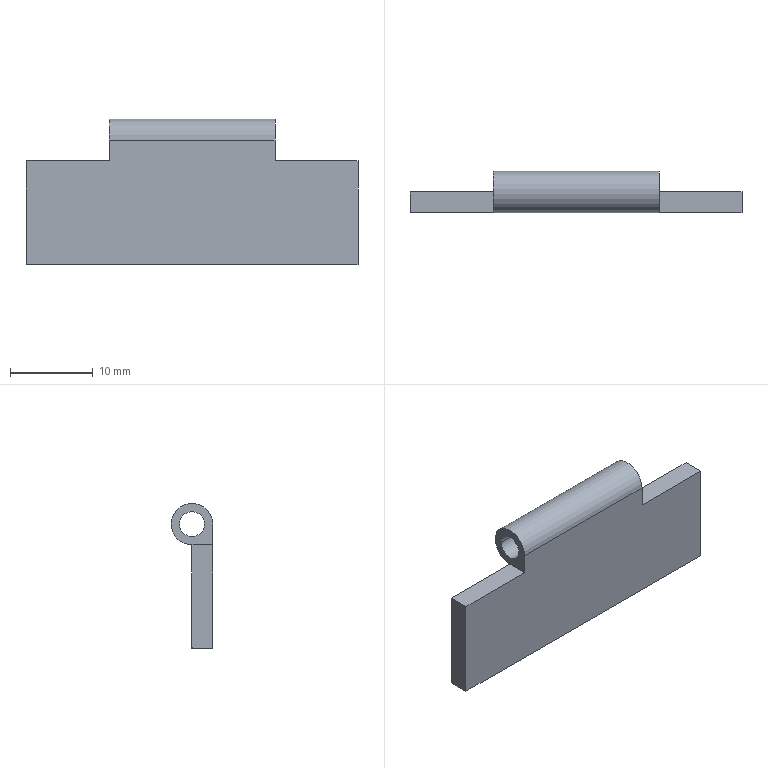Component | SolidWorks | ButtonStation-1_Hinge2-1 | 1 solid | 13 faces | box 40 x 5 x 17.5 mm | volume 1528 mm3 | plane 9 | cylinder 4 | commonest cylinder face diameters 5 x2 3 x2 | material Plain Carbon Steel
STEP:
#1=COLOUR_RGB('',0.7922,0.8196,0.9333);
#2=FILL_AREA_STYLE_COLOUR('',#1);
#3=FILL_AREA_STYLE('',(#2));
#4=SURFACE_STYLE_FILL_AREA(#3);
#5=SURFACE_SIDE_STYLE('',(#4));
#6=SURFACE_STYLE_USAGE(.BOTH.,#5);
#7=PRESENTATION_STYLE_ASSIGNMENT((#6));
#8=CARTESIAN_POINT('',(6.339,24.705,26.713));
#9=VERTEX_POINT('',#8);
#10=CARTESIAN_POINT('',(6.339,24.902,26.713));
#11=VERTEX_POINT('',#10);
#12=CARTESIAN_POINT('',(6.339,24.803,26.713));
#13=DIRECTION('',(-1.,-0.,-0.));
#14=DIRECTION('',(0.,1.,0.));
#15=AXIS2_PLACEMENT_3D('',#12,#13,#14);
#16=CIRCLE('',#15,0.09843);
#17=EDGE_CURVE('',#9,#11,#16,.T.);
#18=ORIENTED_EDGE('',*,*,#17,.T.);
#19=CARTESIAN_POINT('',(5.551,24.902,26.713));
#20=VERTEX_POINT('',#19);
#21=CARTESIAN_POINT('',(6.732,24.902,26.713));
#22=DIRECTION('',(-1.,-0.,-0.));
#23=VECTOR('',#22,39.37);
#24=LINE('',#21,#23);
#25=EDGE_CURVE('',#11,#20,#24,.T.);
#26=ORIENTED_EDGE('',*,*,#25,.T.);
#27=CARTESIAN_POINT('',(5.551,24.705,26.713));
#28=VERTEX_POINT('',#27);
#29=CARTESIAN_POINT('',(5.551,24.803,26.713));
#30=DIRECTION('',(1.,0.,0.));
#31=DIRECTION('',(0.,1.,0.));
#32=AXIS2_PLACEMENT_3D('',#29,#30,#31);
#33=CIRCLE('',#32,0.09843);
#34=EDGE_CURVE('',#20,#28,#33,.T.);
#35=ORIENTED_EDGE('',*,*,#34,.T.);
#36=CARTESIAN_POINT('',(6.732,24.705,26.713));
#37=DIRECTION('',(-1.,-0.,-0.));
#38=VECTOR('',#37,39.37);
#39=LINE('',#36,#38);
#40=EDGE_CURVE('',#9,#28,#39,.T.);
#41=ORIENTED_EDGE('',*,*,#40,.F.);
#42=EDGE_LOOP('',(#18,#26,#35,#41));
#43=FACE_OUTER_BOUND('',#42,.T.);
#44=CARTESIAN_POINT('',(6.732,24.803,26.713));
#45=DIRECTION('',(-1.,-0.,-0.));
#46=DIRECTION('',(0.,1.,0.));
#47=AXIS2_PLACEMENT_3D('',#44,#45,#46);
#48=CYLINDRICAL_SURFACE('',#47,0.09843);
#49=ADVANCED_FACE('',(#43),#48,.T.);
#50=CARTESIAN_POINT('',(6.339,24.862,26.713));
#51=VERTEX_POINT('',#50);
#52=CARTESIAN_POINT('',(6.339,24.744,26.713));
#53=VERTEX_POINT('',#52);
#54=CARTESIAN_POINT('',(6.339,24.803,26.713));
#55=DIRECTION('',(1.,0.,0.));
#56=DIRECTION('',(0.,1.,0.));
#57=AXIS2_PLACEMENT_3D('',#54,#55,#56);
#58=CIRCLE('',#57,0.05906);
#59=EDGE_CURVE('',#51,#53,#58,.T.);
#60=ORIENTED_EDGE('',*,*,#59,.T.);
#61=CARTESIAN_POINT('',(5.551,24.744,26.713));
#62=VERTEX_POINT('',#61);
#63=CARTESIAN_POINT('',(6.732,24.744,26.713));
#64=DIRECTION('',(-1.,-0.,-0.));
#65=VECTOR('',#64,39.37);
#66=LINE('',#63,#65);
#67=EDGE_CURVE('',#53,#62,#66,.T.);
#68=ORIENTED_EDGE('',*,*,#67,.T.);
#69=CARTESIAN_POINT('',(5.551,24.862,26.713));
#70=VERTEX_POINT('',#69);
#71=CARTESIAN_POINT('',(5.551,24.803,26.713));
#72=DIRECTION('',(-1.,-0.,-0.));
#73=DIRECTION('',(0.,1.,0.));
#74=AXIS2_PLACEMENT_3D('',#71,#72,#73);
#75=CIRCLE('',#74,0.05906);
#76=EDGE_CURVE('',#62,#70,#75,.T.);
#77=ORIENTED_EDGE('',*,*,#76,.T.);
#78=CARTESIAN_POINT('',(6.732,24.862,26.713));
#79=DIRECTION('',(-1.,-0.,-0.));
#80=VECTOR('',#79,39.37);
#81=LINE('',#78,#80);
#82=EDGE_CURVE('',#51,#70,#81,.T.);
#83=ORIENTED_EDGE('',*,*,#82,.F.);
#84=EDGE_LOOP('',(#60,#68,#77,#83));
#85=FACE_OUTER_BOUND('',#84,.T.);
#86=CARTESIAN_POINT('',(6.732,24.803,26.713));
#87=DIRECTION('',(-1.,-0.,-0.));
#88=DIRECTION('',(0.,1.,0.));
#89=AXIS2_PLACEMENT_3D('',#86,#87,#88);
#90=CYLINDRICAL_SURFACE('',#89,0.05906);
#91=ADVANCED_FACE('',(#85),#90,.F.);
#92=CARTESIAN_POINT('',(6.339,24.705,26.614));
#93=VERTEX_POINT('',#92);
#94=CARTESIAN_POINT('',(6.339,24.705,27.065));
#95=DIRECTION('',(-0.,0.,1.));
#96=VECTOR('',#95,39.37);
#97=LINE('',#94,#96);
#98=EDGE_CURVE('',#93,#9,#97,.T.);
#99=ORIENTED_EDGE('',*,*,#98,.T.);
#100=ORIENTED_EDGE('',*,*,#40,.T.);
#101=CARTESIAN_POINT('',(5.551,24.705,26.614));
#102=VERTEX_POINT('',#101);
#103=CARTESIAN_POINT('',(5.551,24.705,27.065));
#104=DIRECTION('',(0.,-0.,-1.));
#105=VECTOR('',#104,39.37);
#106=LINE('',#103,#105);
#107=EDGE_CURVE('',#28,#102,#106,.T.);
#108=ORIENTED_EDGE('',*,*,#107,.T.);
#109=CARTESIAN_POINT('',(5.157,24.705,26.614));
#110=VERTEX_POINT('',#109);
#111=CARTESIAN_POINT('',(6.732,24.705,26.614));
#112=DIRECTION('',(-1.,-0.,-0.));
#113=VECTOR('',#112,39.37);
#114=LINE('',#111,#113);
#115=EDGE_CURVE('',#102,#110,#114,.T.);
#116=ORIENTED_EDGE('',*,*,#115,.T.);
#117=CARTESIAN_POINT('',(5.157,24.705,26.122));
#118=VERTEX_POINT('',#117);
#119=CARTESIAN_POINT('',(5.157,24.705,27.065));
#120=DIRECTION('',(0.,-0.,-1.));
#121=VECTOR('',#120,39.37);
#122=LINE('',#119,#121);
#123=EDGE_CURVE('',#110,#118,#122,.T.);
#124=ORIENTED_EDGE('',*,*,#123,.T.);
#125=CARTESIAN_POINT('',(6.732,24.705,26.122));
#126=VERTEX_POINT('',#125);
#127=CARTESIAN_POINT('',(6.732,24.705,26.122));
#128=DIRECTION('',(1.,0.,0.));
#129=VECTOR('',#128,39.37);
#130=LINE('',#127,#129);
#131=EDGE_CURVE('',#118,#126,#130,.T.);
#132=ORIENTED_EDGE('',*,*,#131,.T.);
#133=CARTESIAN_POINT('',(6.732,24.705,26.614));
#134=VERTEX_POINT('',#133);
#135=CARTESIAN_POINT('',(6.732,24.705,27.065));
#136=DIRECTION('',(-0.,0.,1.));
#137=VECTOR('',#136,39.37);
#138=LINE('',#135,#137);
#139=EDGE_CURVE('',#126,#134,#138,.T.);
#140=ORIENTED_EDGE('',*,*,#139,.T.);
#141=CARTESIAN_POINT('',(6.732,24.705,26.614));
#142=DIRECTION('',(-1.,-0.,-0.));
#143=VECTOR('',#142,39.37);
#144=LINE('',#141,#143);
#145=EDGE_CURVE('',#134,#93,#144,.T.);
#146=ORIENTED_EDGE('',*,*,#145,.T.);
#147=EDGE_LOOP('',(#99,#100,#108,#116,#124,#132,#140,#146));
#148=FACE_OUTER_BOUND('',#147,.T.);
#149=CARTESIAN_POINT('',(6.732,24.705,27.065));
#150=DIRECTION('',(0.,-1.,0.));
#151=DIRECTION('',(-0.,0.,1.));
#152=AXIS2_PLACEMENT_3D('',#149,#150,#151);
#153=PLANE('',#152);
#154=ADVANCED_FACE('',(#148),#153,.T.);
#155=ORIENTED_EDGE('',*,*,#25,.F.);
#156=CARTESIAN_POINT('',(6.339,24.803,26.614));
#157=VERTEX_POINT('',#156);
#158=CARTESIAN_POINT('',(6.339,24.803,26.713));
#159=DIRECTION('',(-1.,-0.,-0.));
#160=DIRECTION('',(0.,1.,0.));
#161=AXIS2_PLACEMENT_3D('',#158,#159,#160);
#162=CIRCLE('',#161,0.09843);
#163=EDGE_CURVE('',#11,#157,#162,.T.);
#164=ORIENTED_EDGE('',*,*,#163,.T.);
#165=CARTESIAN_POINT('',(5.551,24.803,26.614));
#166=VERTEX_POINT('',#165);
#167=CARTESIAN_POINT('',(6.732,24.803,26.614));
#168=DIRECTION('',(-1.,-0.,-0.));
#169=VECTOR('',#168,39.37);
#170=LINE('',#167,#169);
#171=EDGE_CURVE('',#157,#166,#170,.T.);
#172=ORIENTED_EDGE('',*,*,#171,.T.);
#173=CARTESIAN_POINT('',(5.551,24.803,26.713));
#174=DIRECTION('',(1.,0.,0.));
#175=DIRECTION('',(0.,1.,-0.));
#176=AXIS2_PLACEMENT_3D('',#173,#174,#175);
#177=CIRCLE('',#176,0.09843);
#178=EDGE_CURVE('',#166,#20,#177,.T.);
#179=ORIENTED_EDGE('',*,*,#178,.T.);
#180=EDGE_LOOP('',(#155,#164,#172,#179));
#181=FACE_OUTER_BOUND('',#180,.T.);
#182=CARTESIAN_POINT('',(6.732,24.803,26.713));
#183=DIRECTION('',(-1.,-0.,-0.));
#184=DIRECTION('',(0.,1.,0.));
#185=AXIS2_PLACEMENT_3D('',#182,#183,#184);
#186=CYLINDRICAL_SURFACE('',#185,0.09843);
#187=ADVANCED_FACE('',(#181),#186,.T.);
#188=ORIENTED_EDGE('',*,*,#98,.F.);
#189=CARTESIAN_POINT('',(6.339,24.902,26.614));
#190=DIRECTION('',(0.,-1.,0.));
#191=VECTOR('',#190,39.37);
#192=LINE('',#189,#191);
#193=EDGE_CURVE('',#157,#93,#192,.T.);
#194=ORIENTED_EDGE('',*,*,#193,.F.);
#195=ORIENTED_EDGE('',*,*,#163,.F.);
#196=ORIENTED_EDGE('',*,*,#17,.F.);
#197=EDGE_LOOP('',(#188,#194,#195,#196));
#198=FACE_OUTER_BOUND('',#197,.T.);
#199=ORIENTED_EDGE('',*,*,#59,.F.);
#200=CARTESIAN_POINT('',(6.339,24.803,26.713));
#201=DIRECTION('',(1.,0.,0.));
#202=DIRECTION('',(0.,1.,0.));
#203=AXIS2_PLACEMENT_3D('',#200,#201,#202);
#204=CIRCLE('',#203,0.05906);
#205=EDGE_CURVE('',#53,#51,#204,.T.);
#206=ORIENTED_EDGE('',*,*,#205,.F.);
#207=EDGE_LOOP('',(#199,#206));
#208=FACE_BOUND('',#207,.T.);
#209=CARTESIAN_POINT('',(6.339,24.902,26.614));
#210=DIRECTION('',(-1.,-0.,-0.));
#211=DIRECTION('',(-0.,1.,-0.));
#212=AXIS2_PLACEMENT_3D('',#209,#210,#211);
#213=PLANE('',#212);
#214=ADVANCED_FACE('',(#198,#208),#213,.F.);
#215=ORIENTED_EDGE('',*,*,#193,.T.);
#216=ORIENTED_EDGE('',*,*,#145,.F.);
#217=CARTESIAN_POINT('',(6.732,24.803,26.614));
#218=VERTEX_POINT('',#217);
#219=CARTESIAN_POINT('',(6.732,24.902,26.614));
#220=DIRECTION('',(0.,-1.,0.));
#221=VECTOR('',#220,39.37);
#222=LINE('',#219,#221);
#223=EDGE_CURVE('',#218,#134,#222,.T.);
#224=ORIENTED_EDGE('',*,*,#223,.F.);
#225=CARTESIAN_POINT('',(6.732,24.803,26.614));
#226=DIRECTION('',(1.,0.,0.));
#227=VECTOR('',#226,39.37);
#228=LINE('',#225,#227);
#229=EDGE_CURVE('',#157,#218,#228,.T.);
#230=ORIENTED_EDGE('',*,*,#229,.F.);
#231=EDGE_LOOP('',(#215,#216,#224,#230));
#232=FACE_OUTER_BOUND('',#231,.T.);
#233=CARTESIAN_POINT('',(6.732,24.902,26.614));
#234=DIRECTION('',(0.,-0.,-1.));
#235=DIRECTION('',(0.,-1.,0.));
#236=AXIS2_PLACEMENT_3D('',#233,#234,#235);
#237=PLANE('',#236);
#238=ADVANCED_FACE('',(#232),#237,.F.);
#239=ORIENTED_EDGE('',*,*,#223,.T.);
#240=ORIENTED_EDGE('',*,*,#139,.F.);
#241=CARTESIAN_POINT('',(6.732,24.803,26.122));
#242=VERTEX_POINT('',#241);
#243=CARTESIAN_POINT('',(6.732,24.765,26.122));
#244=DIRECTION('',(0.,-1.,0.));
#245=VECTOR('',#244,39.37);
#246=LINE('',#243,#245);
#247=EDGE_CURVE('',#242,#126,#246,.T.);
#248=ORIENTED_EDGE('',*,*,#247,.F.);
#249=CARTESIAN_POINT('',(6.732,24.803,27.065));
#250=DIRECTION('',(0.,-0.,-1.));
#251=VECTOR('',#250,39.37);
#252=LINE('',#249,#251);
#253=EDGE_CURVE('',#218,#242,#252,.T.);
#254=ORIENTED_EDGE('',*,*,#253,.F.);
#255=EDGE_LOOP('',(#239,#240,#248,#254));
#256=FACE_OUTER_BOUND('',#255,.T.);
#257=CARTESIAN_POINT('',(6.732,24.765,27.065));
#258=DIRECTION('',(-1.,-0.,-0.));
#259=DIRECTION('',(-0.,1.,-0.));
#260=AXIS2_PLACEMENT_3D('',#257,#258,#259);
#261=PLANE('',#260);
#262=ADVANCED_FACE('',(#256),#261,.F.);
#263=ORIENTED_EDGE('',*,*,#247,.T.);
#264=ORIENTED_EDGE('',*,*,#131,.F.);
#265=CARTESIAN_POINT('',(5.157,24.803,26.122));
#266=VERTEX_POINT('',#265);
#267=CARTESIAN_POINT('',(5.157,24.765,26.122));
#268=DIRECTION('',(-0.,1.,-0.));
#269=VECTOR('',#268,39.37);
#270=LINE('',#267,#269);
#271=EDGE_CURVE('',#118,#266,#270,.T.);
#272=ORIENTED_EDGE('',*,*,#271,.T.);
#273=CARTESIAN_POINT('',(6.732,24.803,26.122));
#274=DIRECTION('',(1.,0.,0.));
#275=VECTOR('',#274,39.37);
#276=LINE('',#273,#275);
#277=EDGE_CURVE('',#266,#242,#276,.T.);
#278=ORIENTED_EDGE('',*,*,#277,.T.);
#279=EDGE_LOOP('',(#263,#264,#272,#278));
#280=FACE_OUTER_BOUND('',#279,.T.);
#281=CARTESIAN_POINT('',(6.732,24.765,26.122));
#282=DIRECTION('',(0.,-0.,-1.));
#283=DIRECTION('',(-1.,-0.,-0.));
#284=AXIS2_PLACEMENT_3D('',#281,#282,#283);
#285=PLANE('',#284);
#286=ADVANCED_FACE('',(#280),#285,.T.);
#287=ORIENTED_EDGE('',*,*,#271,.F.);
#288=ORIENTED_EDGE('',*,*,#123,.F.);
#289=CARTESIAN_POINT('',(5.157,24.803,26.614));
#290=VERTEX_POINT('',#289);
#291=CARTESIAN_POINT('',(5.157,24.765,26.614));
#292=DIRECTION('',(-0.,1.,-0.));
#293=VECTOR('',#292,39.37);
#294=LINE('',#291,#293);
#295=EDGE_CURVE('',#110,#290,#294,.T.);
#296=ORIENTED_EDGE('',*,*,#295,.T.);
#297=CARTESIAN_POINT('',(5.157,24.803,27.065));
#298=DIRECTION('',(0.,-0.,-1.));
#299=VECTOR('',#298,39.37);
#300=LINE('',#297,#299);
#301=EDGE_CURVE('',#290,#266,#300,.T.);
#302=ORIENTED_EDGE('',*,*,#301,.T.);
#303=EDGE_LOOP('',(#287,#288,#296,#302));
#304=FACE_OUTER_BOUND('',#303,.T.);
#305=CARTESIAN_POINT('',(5.157,24.765,27.065));
#306=DIRECTION('',(-1.,-0.,-0.));
#307=DIRECTION('',(-0.,1.,-0.));
#308=AXIS2_PLACEMENT_3D('',#305,#306,#307);
#309=PLANE('',#308);
#310=ADVANCED_FACE('',(#304),#309,.T.);
#311=ORIENTED_EDGE('',*,*,#295,.F.);
#312=ORIENTED_EDGE('',*,*,#115,.F.);
#313=CARTESIAN_POINT('',(5.551,24.902,26.614));
#314=DIRECTION('',(0.,-1.,0.));
#315=VECTOR('',#314,39.37);
#316=LINE('',#313,#315);
#317=EDGE_CURVE('',#166,#102,#316,.T.);
#318=ORIENTED_EDGE('',*,*,#317,.F.);
#319=CARTESIAN_POINT('',(5.157,24.803,26.614));
#320=DIRECTION('',(1.,0.,0.));
#321=VECTOR('',#320,39.37);
#322=LINE('',#319,#321);
#323=EDGE_CURVE('',#290,#166,#322,.T.);
#324=ORIENTED_EDGE('',*,*,#323,.F.);
#325=EDGE_LOOP('',(#311,#312,#318,#324));
#326=FACE_OUTER_BOUND('',#325,.T.);
#327=CARTESIAN_POINT('',(5.157,24.902,26.614));
#328=DIRECTION('',(0.,-0.,-1.));
#329=DIRECTION('',(0.,-1.,0.));
#330=AXIS2_PLACEMENT_3D('',#327,#328,#329);
#331=PLANE('',#330);
#332=ADVANCED_FACE('',(#326),#331,.F.);
#333=ORIENTED_EDGE('',*,*,#107,.F.);
#334=ORIENTED_EDGE('',*,*,#34,.F.);
#335=ORIENTED_EDGE('',*,*,#178,.F.);
#336=ORIENTED_EDGE('',*,*,#317,.T.);
#337=EDGE_LOOP('',(#333,#334,#335,#336));
#338=FACE_OUTER_BOUND('',#337,.T.);
#339=CARTESIAN_POINT('',(5.551,24.803,26.713));
#340=DIRECTION('',(-1.,-0.,-0.));
#341=DIRECTION('',(0.,1.,0.));
#342=AXIS2_PLACEMENT_3D('',#339,#340,#341);
#343=CIRCLE('',#342,0.05906);
#344=EDGE_CURVE('',#70,#62,#343,.T.);
#345=ORIENTED_EDGE('',*,*,#344,.F.);
#346=ORIENTED_EDGE('',*,*,#76,.F.);
#347=EDGE_LOOP('',(#345,#346));
#348=FACE_BOUND('',#347,.T.);
#349=CARTESIAN_POINT('',(5.551,24.902,26.811));
#350=DIRECTION('',(1.,0.,0.));
#351=DIRECTION('',(0.,-1.,0.));
#352=AXIS2_PLACEMENT_3D('',#349,#350,#351);
#353=PLANE('',#352);
#354=ADVANCED_FACE('',(#338,#348),#353,.F.);
#355=ORIENTED_EDGE('',*,*,#67,.F.);
#356=ORIENTED_EDGE('',*,*,#205,.T.);
#357=ORIENTED_EDGE('',*,*,#82,.T.);
#358=ORIENTED_EDGE('',*,*,#344,.T.);
#359=EDGE_LOOP('',(#355,#356,#357,#358));
#360=FACE_OUTER_BOUND('',#359,.T.);
#361=CARTESIAN_POINT('',(6.732,24.803,26.713));
#362=DIRECTION('',(-1.,-0.,-0.));
#363=DIRECTION('',(0.,1.,0.));
#364=AXIS2_PLACEMENT_3D('',#361,#362,#363);
#365=CYLINDRICAL_SURFACE('',#364,0.05906);
#366=ADVANCED_FACE('',(#360),#365,.F.);
#367=ORIENTED_EDGE('',*,*,#253,.T.);
#368=ORIENTED_EDGE('',*,*,#277,.F.);
#369=ORIENTED_EDGE('',*,*,#301,.F.);
#370=ORIENTED_EDGE('',*,*,#323,.T.);
#371=ORIENTED_EDGE('',*,*,#171,.F.);
#372=ORIENTED_EDGE('',*,*,#229,.T.);
#373=EDGE_LOOP('',(#367,#368,#369,#370,#371,#372));
#374=FACE_OUTER_BOUND('',#373,.T.);
#375=CARTESIAN_POINT('',(6.732,24.803,27.065));
#376=DIRECTION('',(-0.,1.,-0.));
#377=DIRECTION('',(1.,0.,0.));
#378=AXIS2_PLACEMENT_3D('',#375,#376,#377);
#379=PLANE('',#378);
#380=ADVANCED_FACE('',(#374),#379,.T.);
#381=CLOSED_SHELL('',(#49,#91,#154,#187,#214,#238,#262,#286,#310,#332,#354,#366,#380));
#382=MANIFOLD_SOLID_BREP('',#381);
#383=STYLED_ITEM('',(#7),#382);
#384=PRESENTATION_LAYER_ASSIGNMENT('','',(#383));
#385=CARTESIAN_POINT('',(0.,0.,0.));
#386=DIRECTION('',(0.,0.,1.));
#387=DIRECTION('',(1.,0.,0.));
#388=AXIS2_PLACEMENT_3D('',#385,#386,#387);
#389=(LENGTH_UNIT()NAMED_UNIT(*)SI_UNIT($,.METRE.));
#390=LENGTH_MEASURE_WITH_UNIT(LENGTH_MEASURE(0.0254),#389);
#391=DIMENSIONAL_EXPONENTS(1.,0.,0.,0.,0.,0.,0.);
#392=(CONVERSION_BASED_UNIT('',#390)LENGTH_UNIT()NAMED_UNIT(#391));
#393=UNCERTAINTY_MEASURE_WITH_UNIT(LENGTH_MEASURE(0.00001),#392,'','');
#394=(NAMED_UNIT(*)PLANE_ANGLE_UNIT()SI_UNIT($,.RADIAN.));
#395=(NAMED_UNIT(*)SI_UNIT($,.STERADIAN.)SOLID_ANGLE_UNIT());
#396=(GEOMETRIC_REPRESENTATION_CONTEXT(3)GLOBAL_UNCERTAINTY_ASSIGNED_CONTEXT((#393))GLOBAL_UNIT_ASSIGNED_CONTEXT((#392,#394,#395))REPRESENTATION_CONTEXT('',''));
#397=ADVANCED_BREP_SHAPE_REPRESENTATION('',(#382,#388),#396);
#398=(LENGTH_UNIT()NAMED_UNIT(*)SI_UNIT($,.METRE.));
#399=LENGTH_MEASURE_WITH_UNIT(LENGTH_MEASURE(0.0254),#398);
#400=DIMENSIONAL_EXPONENTS(1.,0.,0.,0.,0.,0.,0.);
#401=(CONVERSION_BASED_UNIT('',#399)LENGTH_UNIT()NAMED_UNIT(#400));
#402=UNCERTAINTY_MEASURE_WITH_UNIT(LENGTH_MEASURE(0.00001),#401,'','');
#403=(NAMED_UNIT(*)PLANE_ANGLE_UNIT()SI_UNIT($,.RADIAN.));
#404=(NAMED_UNIT(*)SI_UNIT($,.STERADIAN.)SOLID_ANGLE_UNIT());
#405=(GEOMETRIC_REPRESENTATION_CONTEXT(3)GLOBAL_UNCERTAINTY_ASSIGNED_CONTEXT((#402))GLOBAL_UNIT_ASSIGNED_CONTEXT((#401,#403,#404))REPRESENTATION_CONTEXT('',''));
#406=MECHANICAL_DESIGN_GEOMETRIC_PRESENTATION_REPRESENTATION('',(#383),#405);